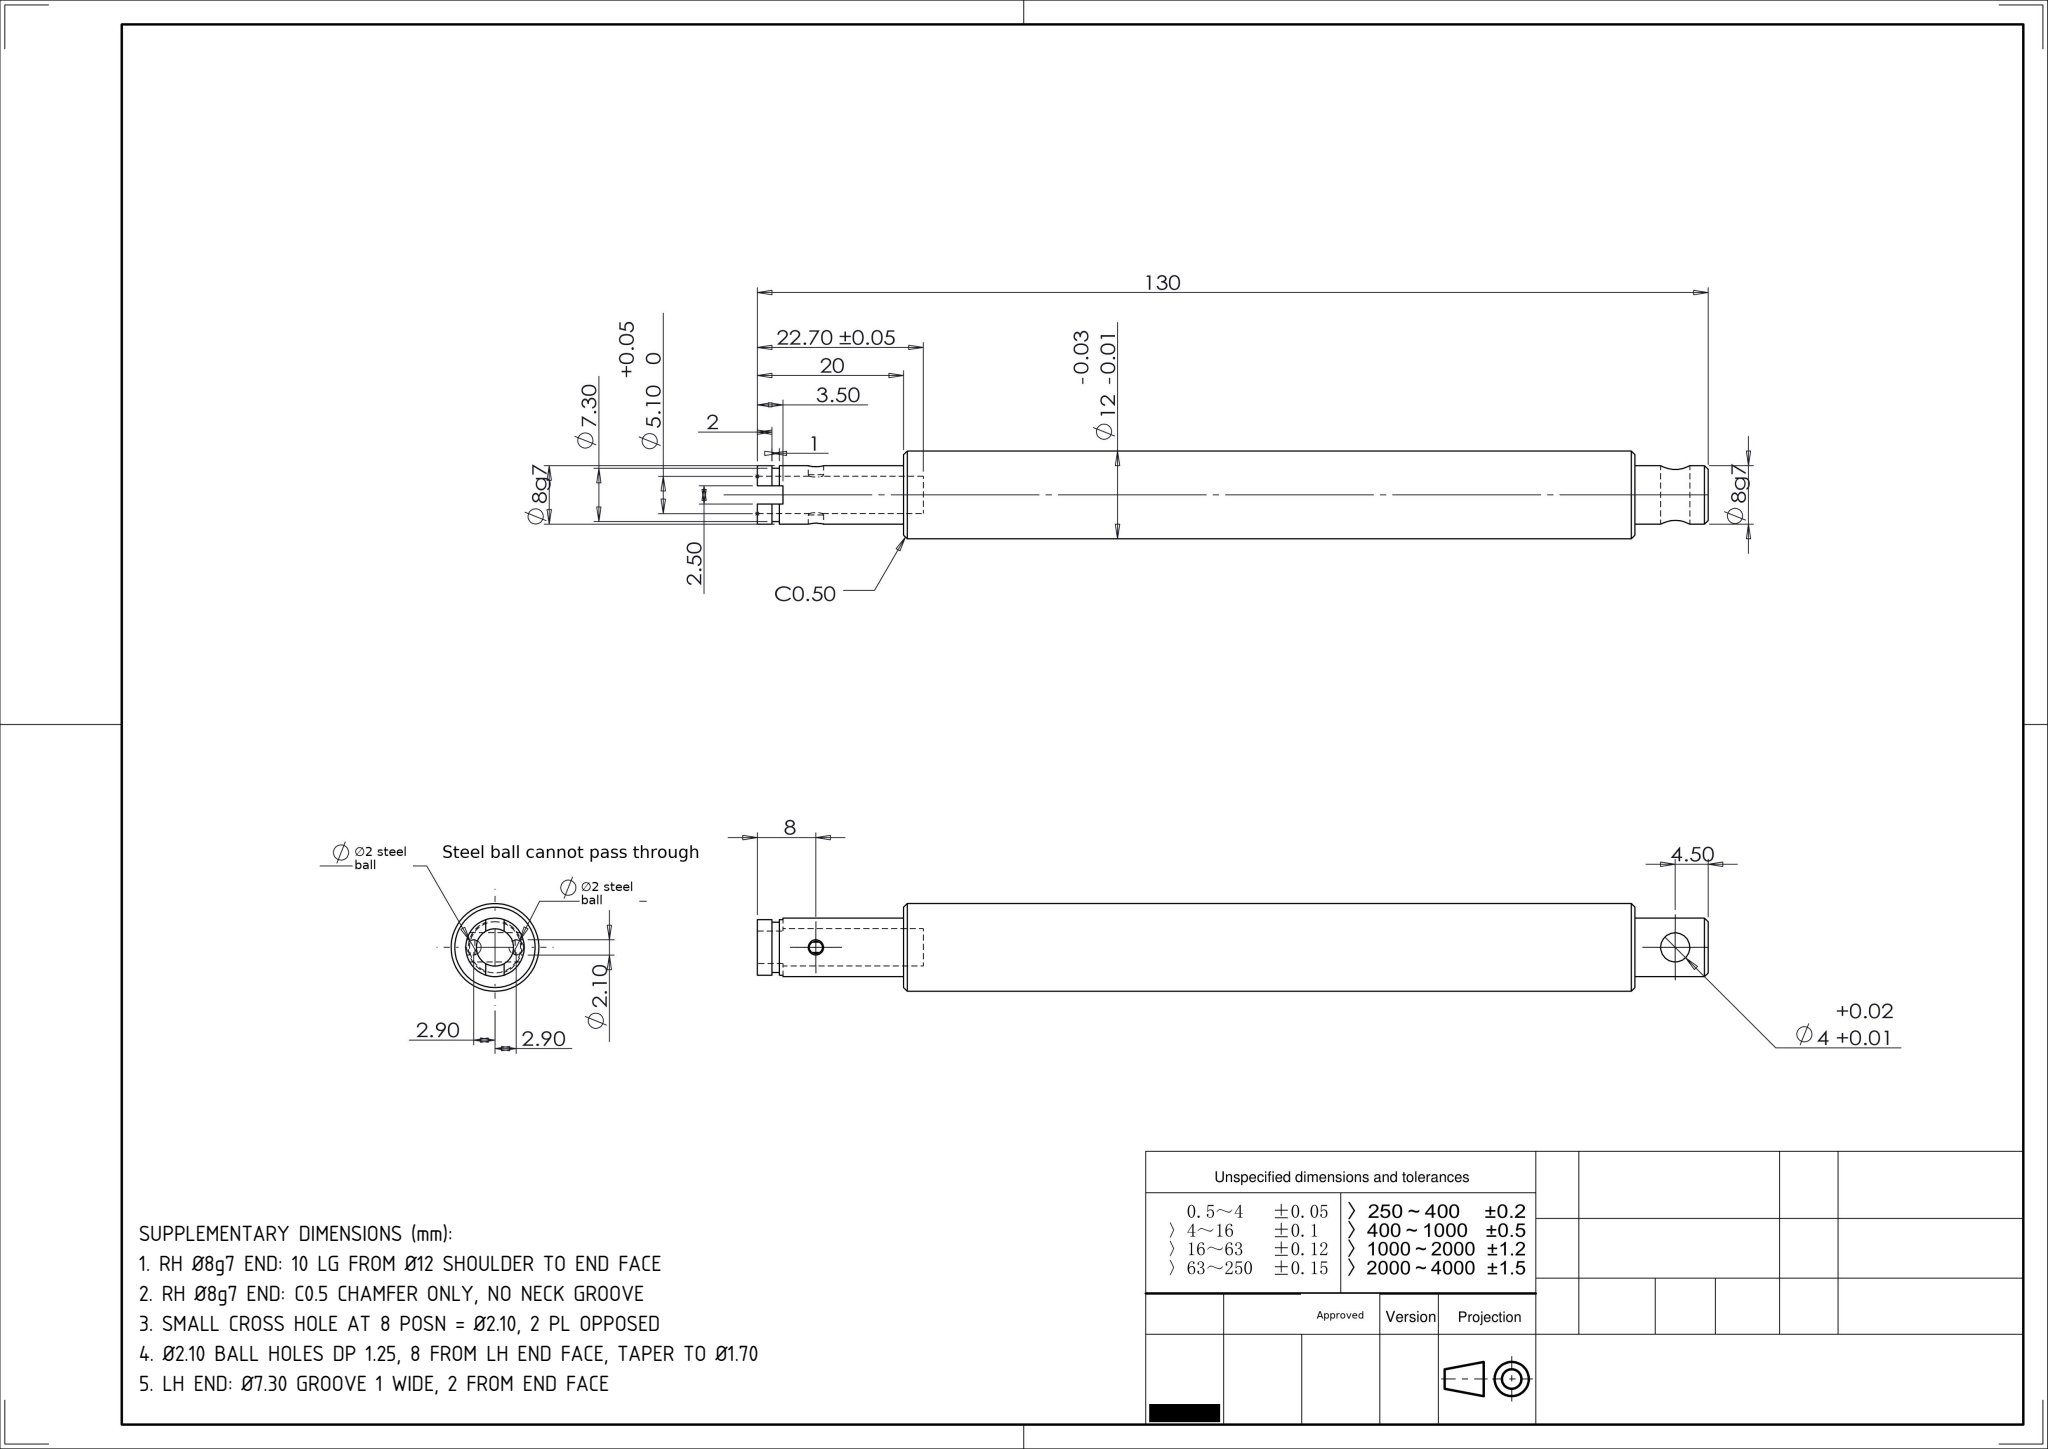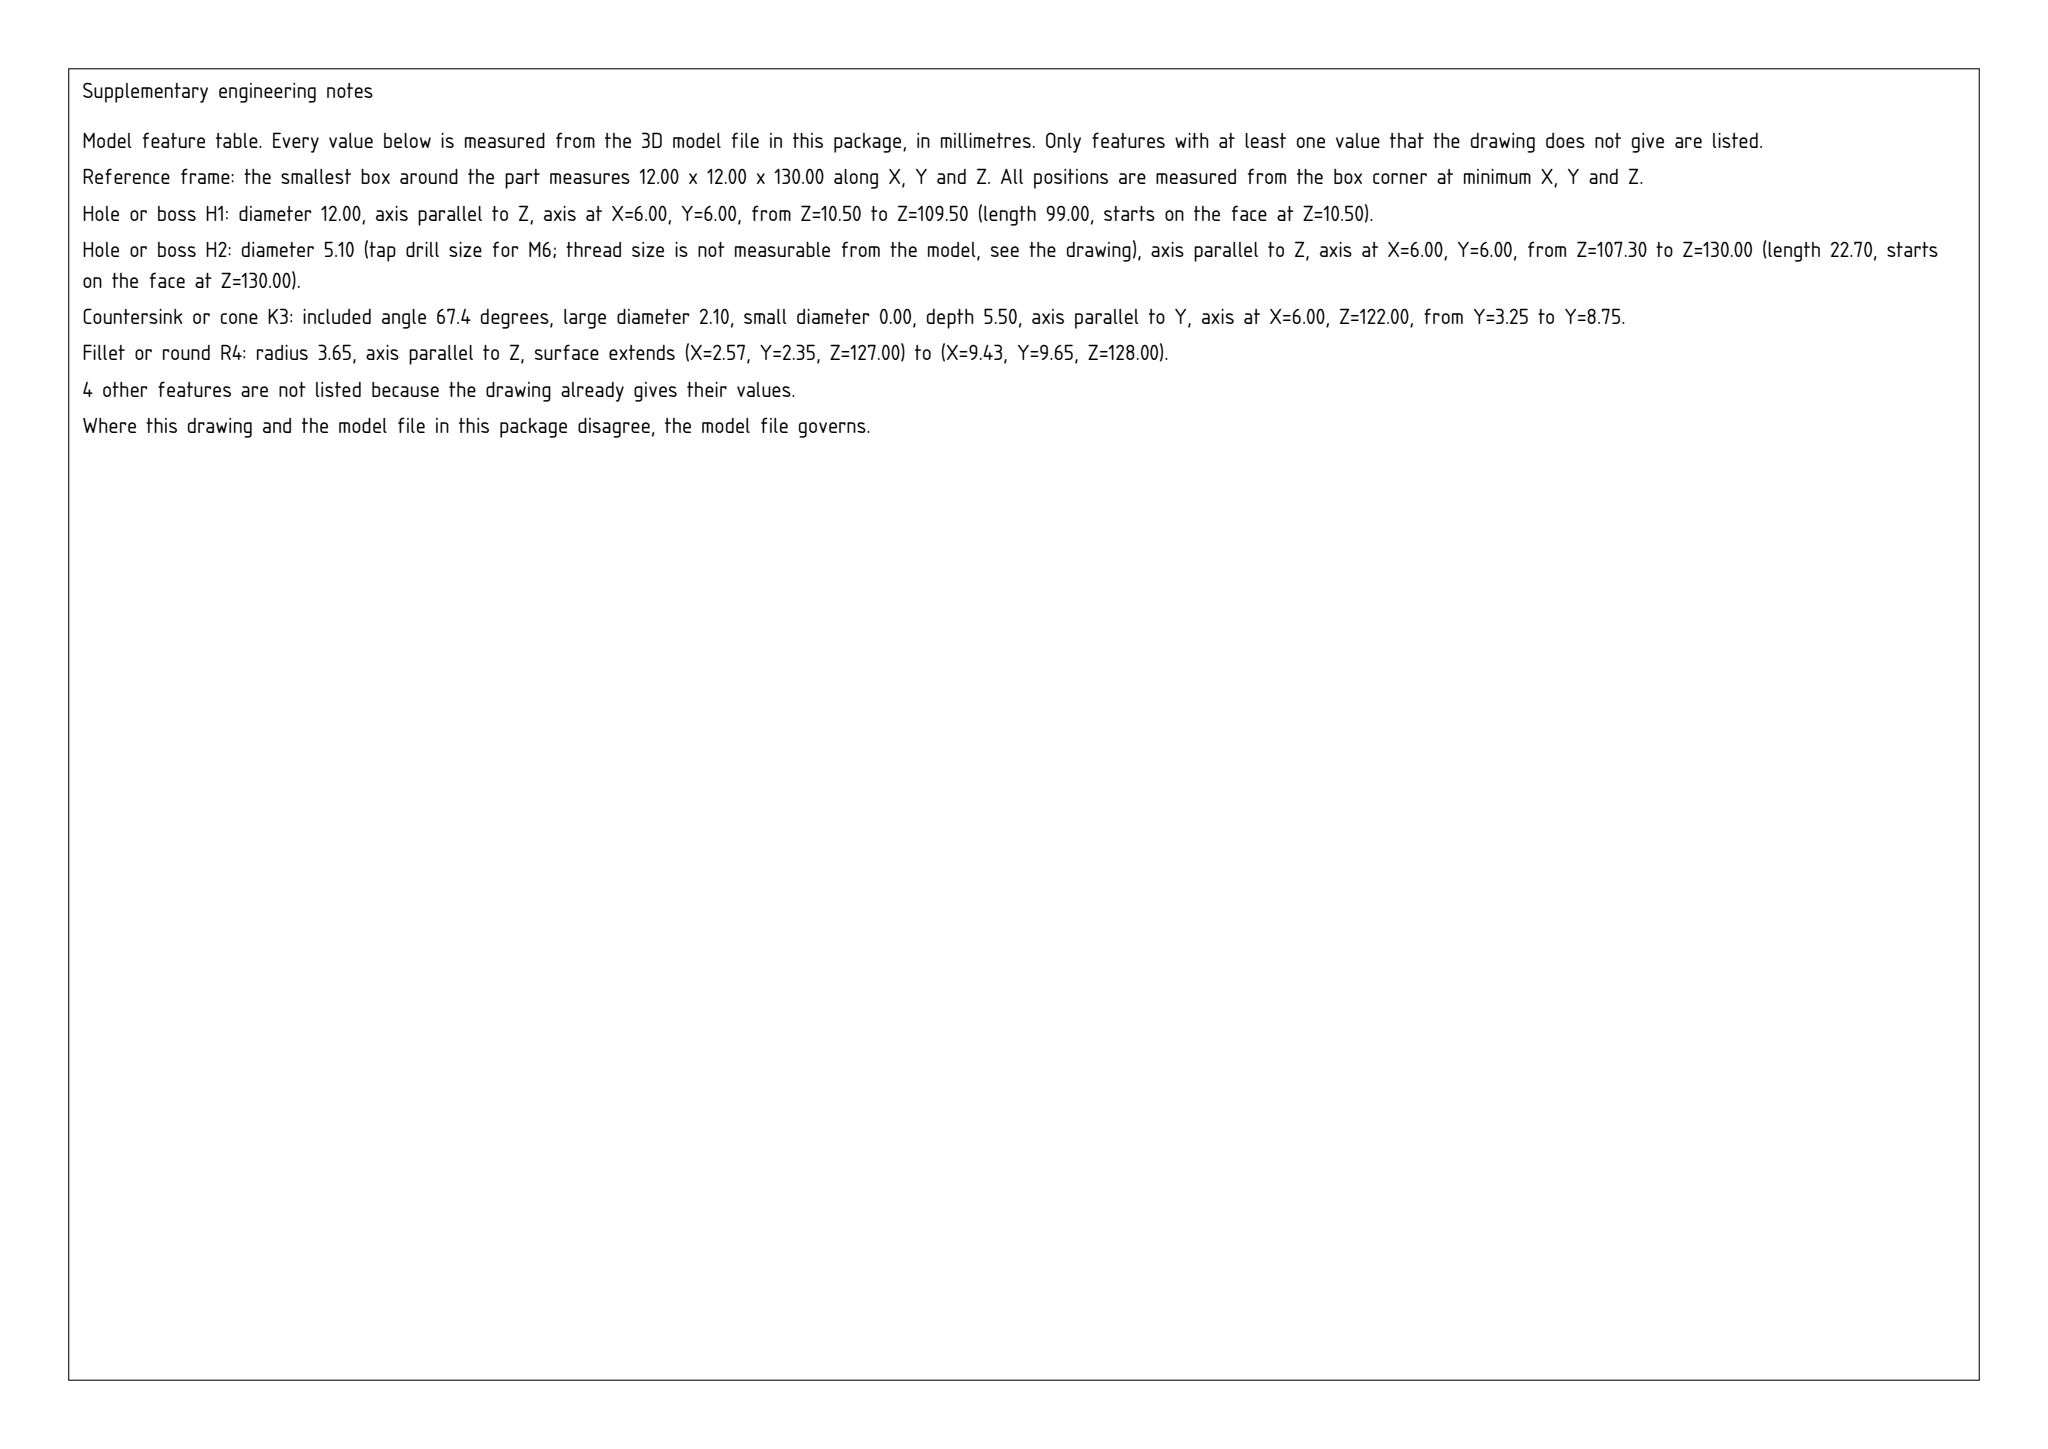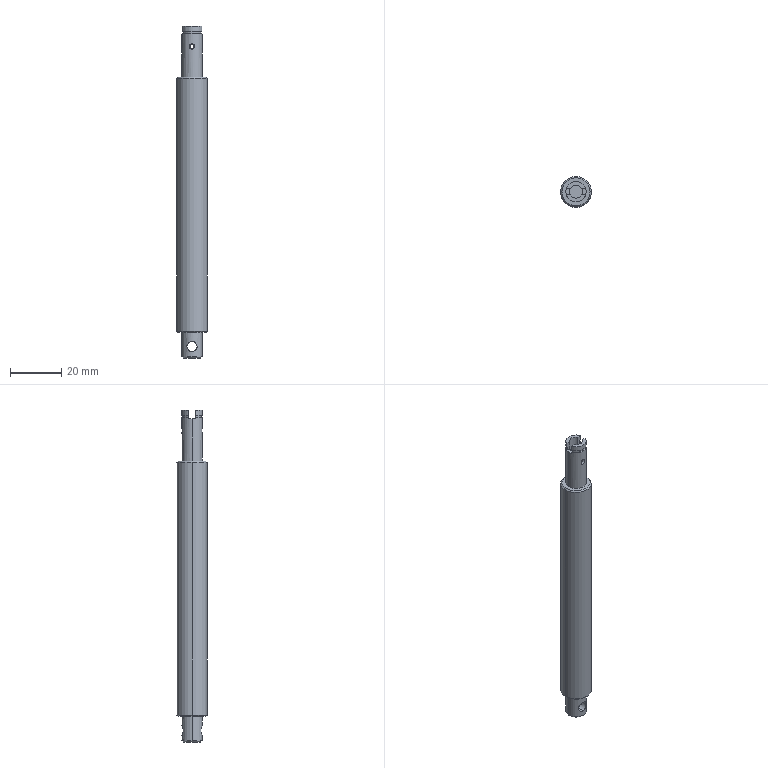Part | SolidWorks | mm | 1 solid | 48 faces | box 12 x 12 x 130 mm | volume 12202 mm3 | plane 20 | cylinder 18 | cone 10 | commonest cylinder face diameters 8 x6 2.1 x4 4 x2 12 x2 5.1 x2 7.3 x2
build123d program:
from build123d import *

# Parameters (mm, degrees)
SKETCH3_W           = 13.415
SKETCH3_H           = 2.5
EXTRUDE3_DEPTH      = 3.5
EXTRUDE4_DEPTH      = 130.455
EXTRUDE4_DEPTH_BACK = 130.455
SKETCH5_R           = 2
CHAMFER1_SIZE       = 0.5
SKETCH6_R           = 11.229
SKETCH6_R_2         = 6
CUT_EXTRUDE1_DEPTH  = 10
CHAMFER2_SIZE       = 0.5


with BuildPart() as part:
    # Sketch1 → Revolve1 (revolve)
    with BuildSketch(Plane(origin=(0, 0, 0), x_dir=(1, 0, 0), z_dir=(0, 1, 0)), mode=Mode.PRIVATE) as revolve1_sk:
        Polygon((-30.056, 122.171), (-30.056, 112.171), (-26.056, 112.171), (-26.056, 110.171), (-28.056, 110.171), (-28.056, 12.171), (-30.056, 12.171), (-30.056, -4.829), (-30.406, -4.829), (-30.406, -5.829), (-30.056, -5.829), (-30.056, -7.829), (-31.506, -7.829), (-31.506, 14.871), (-34.056, 14.871), (-34.056, 122.171), align=None)
    revolve(revolve1_sk.sketch.rotate(Axis((-34.056, 0, -29.69), (0, 0, 1)), 180), axis=Axis((-34.056, 0, -29.69), (0, 0, 1)))

    # Sketch3 → Extrude3 (cut)
    with BuildSketch(Plane.XY.offset(7.829)):
        with Locations((-34.201, 0)):
            Rectangle(SKETCH3_W, SKETCH3_H)
    extrude(amount=-EXTRUDE3_DEPTH, mode=Mode.SUBTRACT)

    # Sketch4 → Cut-Revolve4 (revolve, cut)
    with BuildSketch(Plane(origin=(-34.056, 0, 0), x_dir=(0, 0, -1), z_dir=(1, 0, 0)), mode=Mode.PRIVATE) as cut_revolve4_sk:
        Polygon((1.221, -4.489), (1.221, -2.75), (1.021, -2.45), (0.1714, -2.45), (0.1714, -4.489), align=None)
        Polygon((1.221, 4.564), (0.1714, 4.564), (0.1714, 2.45), (1.021, 2.45), (1.221, 2.75), align=None)
    revolve(cut_revolve4_sk.sketch.rotate(Axis((-34.056, 6.692, -0.1714), (0, -1, 0)), 270), axis=Axis((-34.056, 6.692, -0.1714), (0, -1, 0)), mode=Mode.SUBTRACT)

    # Sketch5 → Extrude4 (cut, two sides: drawn at the far end of the back side and taken through both)
    with BuildSketch(Plane(origin=(0, 0, 0), x_dir=(1, 0, 0), z_dir=(0, 1, 0)).offset(-EXTRUDE4_DEPTH_BACK)):
        with Locations(Location((-34.056, 117.671, 0), (0, 0, 270))):
            Circle(SKETCH5_R)
    extrude(amount=EXTRUDE4_DEPTH + EXTRUDE4_DEPTH_BACK, mode=Mode.SUBTRACT)

    # Chamfer1
    chamfer1_edges = [part.edges().sort_by_distance(p)[0] for p in [
        (-30.056, 0, -122.171),
        (-28.056, 0, -12.171),
    ]]
    chamfer(chamfer1_edges, length=CHAMFER1_SIZE)

    # Sketch6 → Cut-Extrude1 (cut)
    with BuildSketch(Plane.XY.offset(-110.171)):
        with Locations((-34.056, 0)):
            Circle(SKETCH6_R)
        with Locations(Location((-34.056, 0, 0), (0, 0, 180))):
            Circle(SKETCH6_R_2, mode=Mode.SUBTRACT)
    extrude(amount=-CUT_EXTRUDE1_DEPTH, mode=Mode.SUBTRACT)

    # Chamfer2
    chamfer2_edges = [part.edges().sort_by_distance(p)[0] for p in [
        (-28.056, 0, -112.171),
    ]]
    chamfer(chamfer2_edges, length=CHAMFER2_SIZE)


solid = part.part